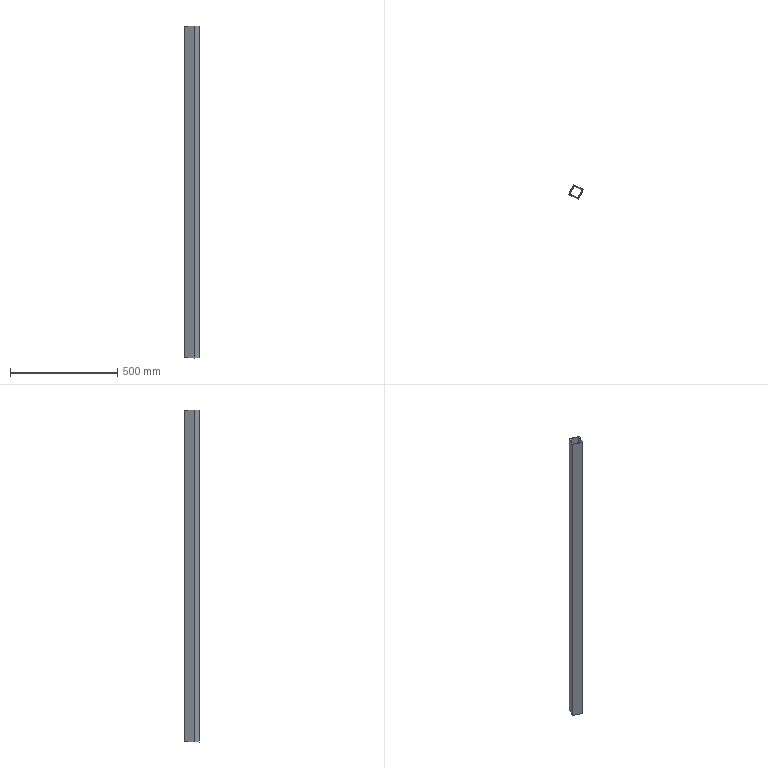Component | SolidWorks | Part40-2 | 1 solid | 10 faces | box 67.2 x 67.2 x 1550 mm | volume 1140800 mm3 | plane 10
STEP:
#1=COLOUR_RGB('',0.7922,0.8196,0.9333);
#2=FILL_AREA_STYLE_COLOUR('',#1);
#3=FILL_AREA_STYLE('',(#2));
#4=SURFACE_STYLE_FILL_AREA(#3);
#5=SURFACE_SIDE_STYLE('',(#4));
#6=SURFACE_STYLE_USAGE(.BOTH.,#5);
#7=PRESENTATION_STYLE_ASSIGNMENT((#6));
#8=CARTESIAN_POINT('',(-55.362,-13.171,102.007));
#9=VERTEX_POINT('',#8);
#10=CARTESIAN_POINT('',(-57.118,-12.281,102.007));
#11=VERTEX_POINT('',#10);
#12=CARTESIAN_POINT('',(-55.362,-13.171,102.007));
#13=DIRECTION('',(-0.892,0.4521,0.));
#14=VECTOR('',#13,39.37);
#15=LINE('',#12,#14);
#16=EDGE_CURVE('',#9,#11,#15,.T.);
#17=ORIENTED_EDGE('',*,*,#16,.T.);
#18=CARTESIAN_POINT('',(-57.118,-12.281,40.983));
#19=VERTEX_POINT('',#18);
#20=CARTESIAN_POINT('',(-57.118,-12.281,40.983));
#21=DIRECTION('',(-0.,-0.,1.));
#22=VECTOR('',#21,39.37);
#23=LINE('',#20,#22);
#24=EDGE_CURVE('',#19,#11,#23,.T.);
#25=ORIENTED_EDGE('',*,*,#24,.F.);
#26=CARTESIAN_POINT('',(-55.362,-13.171,40.983));
#27=VERTEX_POINT('',#26);
#28=CARTESIAN_POINT('',(-55.362,-13.171,40.983));
#29=DIRECTION('',(-0.892,0.4521,0.));
#30=VECTOR('',#29,39.37);
#31=LINE('',#28,#30);
#32=EDGE_CURVE('',#27,#19,#31,.T.);
#33=ORIENTED_EDGE('',*,*,#32,.F.);
#34=CARTESIAN_POINT('',(-55.362,-13.171,40.983));
#35=DIRECTION('',(-0.,-0.,1.));
#36=VECTOR('',#35,39.37);
#37=LINE('',#34,#36);
#38=EDGE_CURVE('',#27,#9,#37,.T.);
#39=ORIENTED_EDGE('',*,*,#38,.T.);
#40=EDGE_LOOP('',(#17,#25,#33,#39));
#41=FACE_OUTER_BOUND('',#40,.T.);
#42=CARTESIAN_POINT('',(-55.362,-13.171,40.983));
#43=DIRECTION('',(0.4521,0.892,0.));
#44=DIRECTION('',(0.892,-0.4521,-0.));
#45=AXIS2_PLACEMENT_3D('',#42,#43,#44);
#46=PLANE('',#45);
#47=ADVANCED_FACE('',(#41),#46,.F.);
#48=CARTESIAN_POINT('',(-56.228,-10.525,102.007));
#49=VERTEX_POINT('',#48);
#50=CARTESIAN_POINT('',(-57.118,-12.281,102.007));
#51=DIRECTION('',(0.4521,0.892,0.));
#52=VECTOR('',#51,39.37);
#53=LINE('',#50,#52);
#54=EDGE_CURVE('',#11,#49,#53,.T.);
#55=ORIENTED_EDGE('',*,*,#54,.T.);
#56=CARTESIAN_POINT('',(-56.228,-10.525,40.983));
#57=VERTEX_POINT('',#56);
#58=CARTESIAN_POINT('',(-56.228,-10.525,40.983));
#59=DIRECTION('',(-0.,-0.,1.));
#60=VECTOR('',#59,39.37);
#61=LINE('',#58,#60);
#62=EDGE_CURVE('',#57,#49,#61,.T.);
#63=ORIENTED_EDGE('',*,*,#62,.F.);
#64=CARTESIAN_POINT('',(-57.118,-12.281,40.983));
#65=DIRECTION('',(0.4521,0.892,0.));
#66=VECTOR('',#65,39.37);
#67=LINE('',#64,#66);
#68=EDGE_CURVE('',#19,#57,#67,.T.);
#69=ORIENTED_EDGE('',*,*,#68,.F.);
#70=ORIENTED_EDGE('',*,*,#24,.T.);
#71=EDGE_LOOP('',(#55,#63,#69,#70));
#72=FACE_OUTER_BOUND('',#71,.T.);
#73=CARTESIAN_POINT('',(-57.118,-12.281,40.983));
#74=DIRECTION('',(0.892,-0.4521,-0.));
#75=DIRECTION('',(-0.4521,-0.892,-0.));
#76=AXIS2_PLACEMENT_3D('',#73,#74,#75);
#77=PLANE('',#76);
#78=ADVANCED_FACE('',(#72),#77,.F.);
#79=CARTESIAN_POINT('',(-54.472,-11.415,102.007));
#80=VERTEX_POINT('',#79);
#81=CARTESIAN_POINT('',(-54.472,-11.415,102.007));
#82=DIRECTION('',(-0.892,0.4521,0.));
#83=VECTOR('',#82,39.37);
#84=LINE('',#81,#83);
#85=EDGE_CURVE('',#80,#49,#84,.T.);
#86=ORIENTED_EDGE('',*,*,#85,.F.);
#87=CARTESIAN_POINT('',(-54.472,-11.415,40.983));
#88=VERTEX_POINT('',#87);
#89=CARTESIAN_POINT('',(-54.472,-11.415,40.983));
#90=DIRECTION('',(-0.,-0.,1.));
#91=VECTOR('',#90,39.37);
#92=LINE('',#89,#91);
#93=EDGE_CURVE('',#88,#80,#92,.T.);
#94=ORIENTED_EDGE('',*,*,#93,.F.);
#95=CARTESIAN_POINT('',(-54.472,-11.415,40.983));
#96=DIRECTION('',(-0.892,0.4521,0.));
#97=VECTOR('',#96,39.37);
#98=LINE('',#95,#97);
#99=EDGE_CURVE('',#88,#57,#98,.T.);
#100=ORIENTED_EDGE('',*,*,#99,.T.);
#101=ORIENTED_EDGE('',*,*,#62,.T.);
#102=EDGE_LOOP('',(#86,#94,#100,#101));
#103=FACE_OUTER_BOUND('',#102,.T.);
#104=CARTESIAN_POINT('',(-54.472,-11.415,40.983));
#105=DIRECTION('',(0.4521,0.892,0.));
#106=DIRECTION('',(0.892,-0.4521,-0.));
#107=AXIS2_PLACEMENT_3D('',#104,#105,#106);
#108=PLANE('',#107);
#109=ADVANCED_FACE('',(#103),#108,.T.);
#110=CARTESIAN_POINT('',(-55.362,-13.171,102.007));
#111=DIRECTION('',(0.4521,0.892,0.));
#112=VECTOR('',#111,39.37);
#113=LINE('',#110,#112);
#114=EDGE_CURVE('',#9,#80,#113,.T.);
#115=ORIENTED_EDGE('',*,*,#114,.F.);
#116=ORIENTED_EDGE('',*,*,#38,.F.);
#117=CARTESIAN_POINT('',(-55.362,-13.171,40.983));
#118=DIRECTION('',(0.4521,0.892,0.));
#119=VECTOR('',#118,39.37);
#120=LINE('',#117,#119);
#121=EDGE_CURVE('',#27,#88,#120,.T.);
#122=ORIENTED_EDGE('',*,*,#121,.T.);
#123=ORIENTED_EDGE('',*,*,#93,.T.);
#124=EDGE_LOOP('',(#115,#116,#122,#123));
#125=FACE_OUTER_BOUND('',#124,.T.);
#126=CARTESIAN_POINT('',(-55.362,-13.171,40.983));
#127=DIRECTION('',(0.892,-0.4521,-0.));
#128=DIRECTION('',(-0.4521,-0.892,-0.));
#129=AXIS2_PLACEMENT_3D('',#126,#127,#128);
#130=PLANE('',#129);
#131=ADVANCED_FACE('',(#125),#130,.T.);
#132=CARTESIAN_POINT('',(-55.431,-12.959,40.983));
#133=VERTEX_POINT('',#132);
#134=CARTESIAN_POINT('',(-56.906,-12.212,40.983));
#135=VERTEX_POINT('',#134);
#136=CARTESIAN_POINT('',(-55.291,-13.031,40.983));
#137=DIRECTION('',(-0.892,0.4521,0.));
#138=VECTOR('',#137,39.37);
#139=LINE('',#136,#138);
#140=EDGE_CURVE('',#133,#135,#139,.T.);
#141=ORIENTED_EDGE('',*,*,#140,.F.);
#142=CARTESIAN_POINT('',(-54.684,-11.484,40.983));
#143=VERTEX_POINT('',#142);
#144=CARTESIAN_POINT('',(-55.502,-13.1,40.983));
#145=DIRECTION('',(0.4521,0.892,0.));
#146=VECTOR('',#145,39.37);
#147=LINE('',#144,#146);
#148=EDGE_CURVE('',#133,#143,#147,.T.);
#149=ORIENTED_EDGE('',*,*,#148,.T.);
#150=CARTESIAN_POINT('',(-56.159,-10.737,40.983));
#151=VERTEX_POINT('',#150);
#152=CARTESIAN_POINT('',(-54.543,-11.556,40.983));
#153=DIRECTION('',(-0.892,0.4521,0.));
#154=VECTOR('',#153,39.37);
#155=LINE('',#152,#154);
#156=EDGE_CURVE('',#143,#151,#155,.T.);
#157=ORIENTED_EDGE('',*,*,#156,.T.);
#158=CARTESIAN_POINT('',(-56.977,-12.352,40.983));
#159=DIRECTION('',(0.4521,0.892,0.));
#160=VECTOR('',#159,39.37);
#161=LINE('',#158,#160);
#162=EDGE_CURVE('',#135,#151,#161,.T.);
#163=ORIENTED_EDGE('',*,*,#162,.F.);
#164=EDGE_LOOP('',(#141,#149,#157,#163));
#165=FACE_BOUND('',#164,.T.);
#166=ORIENTED_EDGE('',*,*,#32,.T.);
#167=ORIENTED_EDGE('',*,*,#68,.T.);
#168=ORIENTED_EDGE('',*,*,#99,.F.);
#169=ORIENTED_EDGE('',*,*,#121,.F.);
#170=EDGE_LOOP('',(#166,#167,#168,#169));
#171=FACE_OUTER_BOUND('',#170,.T.);
#172=CARTESIAN_POINT('',(-54.99,-11.459,40.983));
#173=DIRECTION('',(0.,0.,-1.));
#174=DIRECTION('',(-0.892,0.4521,0.));
#175=AXIS2_PLACEMENT_3D('',#172,#173,#174);
#176=PLANE('',#175);
#177=ADVANCED_FACE('',(#165,#171),#176,.T.);
#178=CARTESIAN_POINT('',(-55.431,-12.959,102.007));
#179=VERTEX_POINT('',#178);
#180=CARTESIAN_POINT('',(-54.684,-11.484,102.007));
#181=VERTEX_POINT('',#180);
#182=CARTESIAN_POINT('',(-55.502,-13.1,102.007));
#183=DIRECTION('',(0.4521,0.892,0.));
#184=VECTOR('',#183,39.37);
#185=LINE('',#182,#184);
#186=EDGE_CURVE('',#179,#181,#185,.T.);
#187=ORIENTED_EDGE('',*,*,#186,.F.);
#188=CARTESIAN_POINT('',(-56.906,-12.212,102.007));
#189=VERTEX_POINT('',#188);
#190=CARTESIAN_POINT('',(-55.291,-13.031,102.007));
#191=DIRECTION('',(-0.892,0.4521,0.));
#192=VECTOR('',#191,39.37);
#193=LINE('',#190,#192);
#194=EDGE_CURVE('',#179,#189,#193,.T.);
#195=ORIENTED_EDGE('',*,*,#194,.T.);
#196=CARTESIAN_POINT('',(-56.159,-10.737,102.007));
#197=VERTEX_POINT('',#196);
#198=CARTESIAN_POINT('',(-56.977,-12.352,102.007));
#199=DIRECTION('',(0.4521,0.892,0.));
#200=VECTOR('',#199,39.37);
#201=LINE('',#198,#200);
#202=EDGE_CURVE('',#189,#197,#201,.T.);
#203=ORIENTED_EDGE('',*,*,#202,.T.);
#204=CARTESIAN_POINT('',(-54.543,-11.556,102.007));
#205=DIRECTION('',(-0.892,0.4521,0.));
#206=VECTOR('',#205,39.37);
#207=LINE('',#204,#206);
#208=EDGE_CURVE('',#181,#197,#207,.T.);
#209=ORIENTED_EDGE('',*,*,#208,.F.);
#210=EDGE_LOOP('',(#187,#195,#203,#209));
#211=FACE_BOUND('',#210,.T.);
#212=ORIENTED_EDGE('',*,*,#16,.F.);
#213=ORIENTED_EDGE('',*,*,#114,.T.);
#214=ORIENTED_EDGE('',*,*,#85,.T.);
#215=ORIENTED_EDGE('',*,*,#54,.F.);
#216=EDGE_LOOP('',(#212,#213,#214,#215));
#217=FACE_OUTER_BOUND('',#216,.T.);
#218=CARTESIAN_POINT('',(-54.99,-11.459,102.007));
#219=DIRECTION('',(0.,0.,-1.));
#220=DIRECTION('',(-0.892,0.4521,0.));
#221=AXIS2_PLACEMENT_3D('',#218,#219,#220);
#222=PLANE('',#221);
#223=ADVANCED_FACE('',(#211,#217),#222,.F.);
#224=ORIENTED_EDGE('',*,*,#194,.F.);
#225=CARTESIAN_POINT('',(-55.431,-12.959,40.983));
#226=DIRECTION('',(-0.,-0.,1.));
#227=VECTOR('',#226,39.37);
#228=LINE('',#225,#227);
#229=EDGE_CURVE('',#133,#179,#228,.T.);
#230=ORIENTED_EDGE('',*,*,#229,.F.);
#231=ORIENTED_EDGE('',*,*,#140,.T.);
#232=CARTESIAN_POINT('',(-56.906,-12.212,40.983));
#233=DIRECTION('',(-0.,-0.,1.));
#234=VECTOR('',#233,39.37);
#235=LINE('',#232,#234);
#236=EDGE_CURVE('',#135,#189,#235,.T.);
#237=ORIENTED_EDGE('',*,*,#236,.T.);
#238=EDGE_LOOP('',(#224,#230,#231,#237));
#239=FACE_OUTER_BOUND('',#238,.T.);
#240=CARTESIAN_POINT('',(-55.291,-13.031,40.983));
#241=DIRECTION('',(0.4521,0.892,0.));
#242=DIRECTION('',(0.892,-0.4521,-0.));
#243=AXIS2_PLACEMENT_3D('',#240,#241,#242);
#244=PLANE('',#243);
#245=ADVANCED_FACE('',(#239),#244,.T.);
#246=ORIENTED_EDGE('',*,*,#202,.F.);
#247=ORIENTED_EDGE('',*,*,#236,.F.);
#248=ORIENTED_EDGE('',*,*,#162,.T.);
#249=CARTESIAN_POINT('',(-56.159,-10.737,40.983));
#250=DIRECTION('',(-0.,-0.,1.));
#251=VECTOR('',#250,39.37);
#252=LINE('',#249,#251);
#253=EDGE_CURVE('',#151,#197,#252,.T.);
#254=ORIENTED_EDGE('',*,*,#253,.T.);
#255=EDGE_LOOP('',(#246,#247,#248,#254));
#256=FACE_OUTER_BOUND('',#255,.T.);
#257=CARTESIAN_POINT('',(-56.977,-12.352,40.983));
#258=DIRECTION('',(0.892,-0.4521,-0.));
#259=DIRECTION('',(-0.4521,-0.892,-0.));
#260=AXIS2_PLACEMENT_3D('',#257,#258,#259);
#261=PLANE('',#260);
#262=ADVANCED_FACE('',(#256),#261,.T.);
#263=ORIENTED_EDGE('',*,*,#208,.T.);
#264=ORIENTED_EDGE('',*,*,#253,.F.);
#265=ORIENTED_EDGE('',*,*,#156,.F.);
#266=CARTESIAN_POINT('',(-54.684,-11.484,40.983));
#267=DIRECTION('',(-0.,-0.,1.));
#268=VECTOR('',#267,39.37);
#269=LINE('',#266,#268);
#270=EDGE_CURVE('',#143,#181,#269,.T.);
#271=ORIENTED_EDGE('',*,*,#270,.T.);
#272=EDGE_LOOP('',(#263,#264,#265,#271));
#273=FACE_OUTER_BOUND('',#272,.T.);
#274=CARTESIAN_POINT('',(-54.543,-11.556,40.983));
#275=DIRECTION('',(0.4521,0.892,0.));
#276=DIRECTION('',(0.892,-0.4521,-0.));
#277=AXIS2_PLACEMENT_3D('',#274,#275,#276);
#278=PLANE('',#277);
#279=ADVANCED_FACE('',(#273),#278,.F.);
#280=ORIENTED_EDGE('',*,*,#186,.T.);
#281=ORIENTED_EDGE('',*,*,#270,.F.);
#282=ORIENTED_EDGE('',*,*,#148,.F.);
#283=ORIENTED_EDGE('',*,*,#229,.T.);
#284=EDGE_LOOP('',(#280,#281,#282,#283));
#285=FACE_OUTER_BOUND('',#284,.T.);
#286=CARTESIAN_POINT('',(-55.502,-13.1,40.983));
#287=DIRECTION('',(0.892,-0.4521,-0.));
#288=DIRECTION('',(-0.4521,-0.892,-0.));
#289=AXIS2_PLACEMENT_3D('',#286,#287,#288);
#290=PLANE('',#289);
#291=ADVANCED_FACE('',(#285),#290,.F.);
#292=CLOSED_SHELL('',(#47,#78,#109,#131,#177,#223,#245,#262,#279,#291));
#293=MANIFOLD_SOLID_BREP('',#292);
#294=STYLED_ITEM('',(#7),#293);
#295=PRESENTATION_LAYER_ASSIGNMENT('','',(#294));
#296=CARTESIAN_POINT('',(0.,0.,0.));
#297=DIRECTION('',(0.,0.,1.));
#298=DIRECTION('',(1.,0.,0.));
#299=AXIS2_PLACEMENT_3D('',#296,#297,#298);
#300=(LENGTH_UNIT()NAMED_UNIT(*)SI_UNIT($,.METRE.));
#301=LENGTH_MEASURE_WITH_UNIT(LENGTH_MEASURE(0.0254),#300);
#302=DIMENSIONAL_EXPONENTS(1.,0.,0.,0.,0.,0.,0.);
#303=(CONVERSION_BASED_UNIT('',#301)LENGTH_UNIT()NAMED_UNIT(#302));
#304=UNCERTAINTY_MEASURE_WITH_UNIT(LENGTH_MEASURE(0.00001),#303,'','');
#305=(NAMED_UNIT(*)PLANE_ANGLE_UNIT()SI_UNIT($,.RADIAN.));
#306=(NAMED_UNIT(*)SI_UNIT($,.STERADIAN.)SOLID_ANGLE_UNIT());
#307=(GEOMETRIC_REPRESENTATION_CONTEXT(3)GLOBAL_UNCERTAINTY_ASSIGNED_CONTEXT((#304))GLOBAL_UNIT_ASSIGNED_CONTEXT((#303,#305,#306))REPRESENTATION_CONTEXT('',''));
#308=ADVANCED_BREP_SHAPE_REPRESENTATION('',(#293,#299),#307);
#309=(LENGTH_UNIT()NAMED_UNIT(*)SI_UNIT($,.METRE.));
#310=LENGTH_MEASURE_WITH_UNIT(LENGTH_MEASURE(0.0254),#309);
#311=DIMENSIONAL_EXPONENTS(1.,0.,0.,0.,0.,0.,0.);
#312=(CONVERSION_BASED_UNIT('',#310)LENGTH_UNIT()NAMED_UNIT(#311));
#313=UNCERTAINTY_MEASURE_WITH_UNIT(LENGTH_MEASURE(0.00001),#312,'','');
#314=(NAMED_UNIT(*)PLANE_ANGLE_UNIT()SI_UNIT($,.RADIAN.));
#315=(NAMED_UNIT(*)SI_UNIT($,.STERADIAN.)SOLID_ANGLE_UNIT());
#316=(GEOMETRIC_REPRESENTATION_CONTEXT(3)GLOBAL_UNCERTAINTY_ASSIGNED_CONTEXT((#313))GLOBAL_UNIT_ASSIGNED_CONTEXT((#312,#314,#315))REPRESENTATION_CONTEXT('',''));
#317=MECHANICAL_DESIGN_GEOMETRIC_PRESENTATION_REPRESENTATION('',(#294),#316);